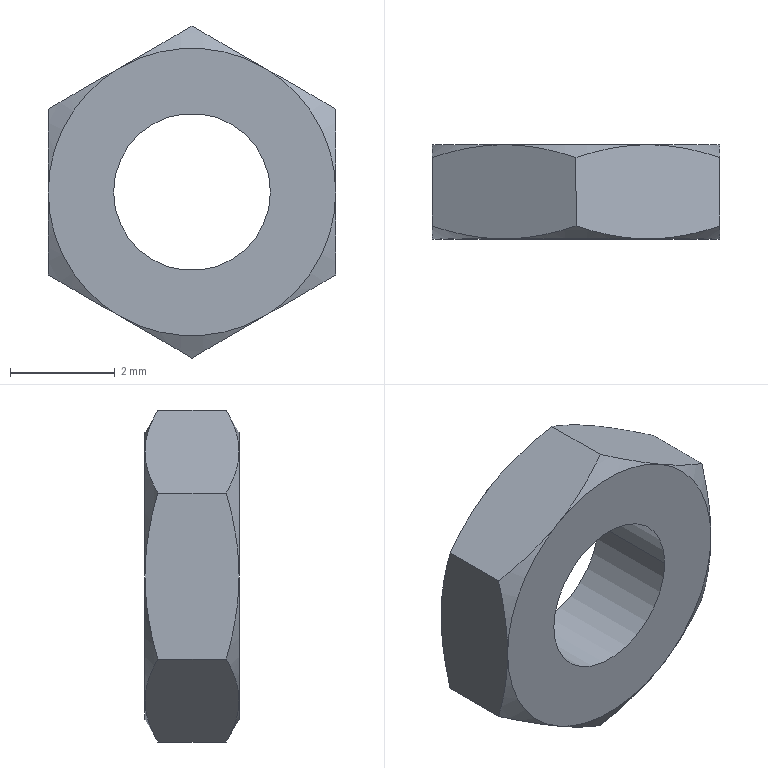Component | NX | HEX_THIN_NUT_A_M3 | 1 solid | 22 faces | volume 34 mm3 | cone 12 | plane 8 | cylinder 2 | commonest cylinder face diameters 3 x2